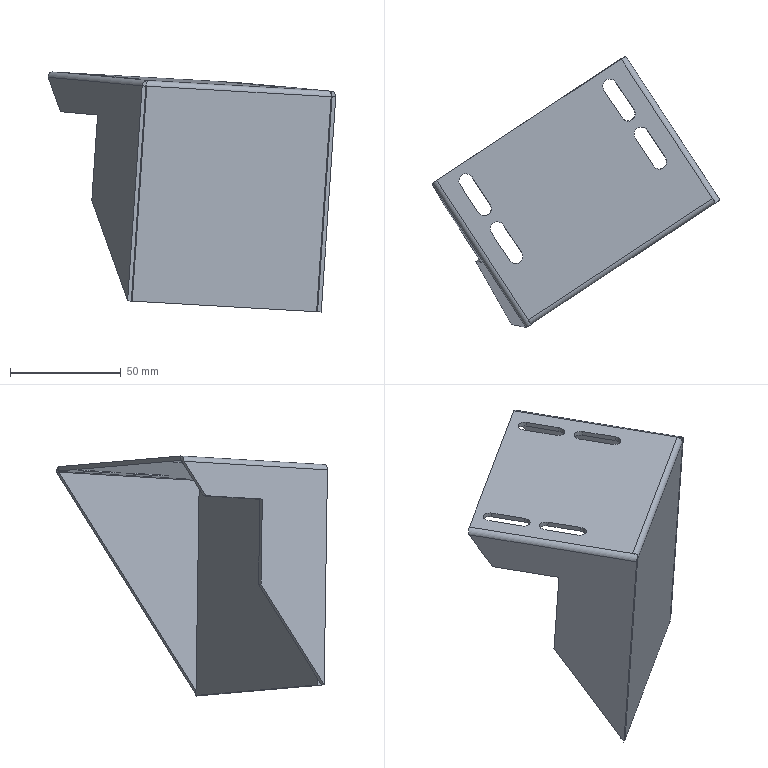Component | SolidWorks | BucketCylinderConnection-1 | 1 solid | 53 faces | volume 48711 mm3 | plane 33 | cylinder 18 | spline 2 | commonest cylinder face diameters 6.5 x12 1 x3 5 x3 | material AISI 304